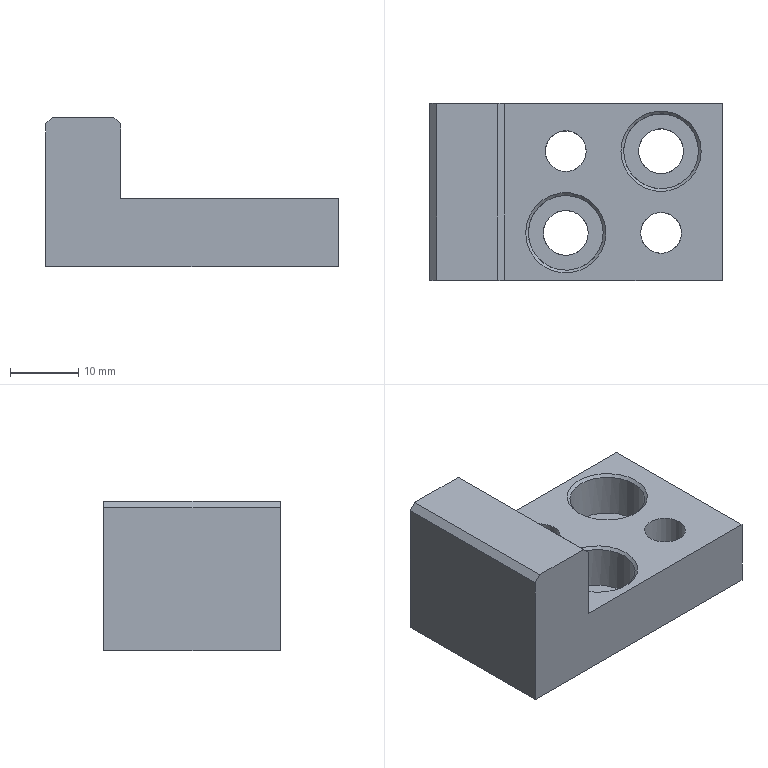Component | NX | TOOL_SETTING_BLOCK | 1 solid | 22 faces | volume 12500 mm3 | plane 12 | cylinder 6 | cone 4 | commonest cylinder face diameters 6 x2 6.6 x2 11 x2